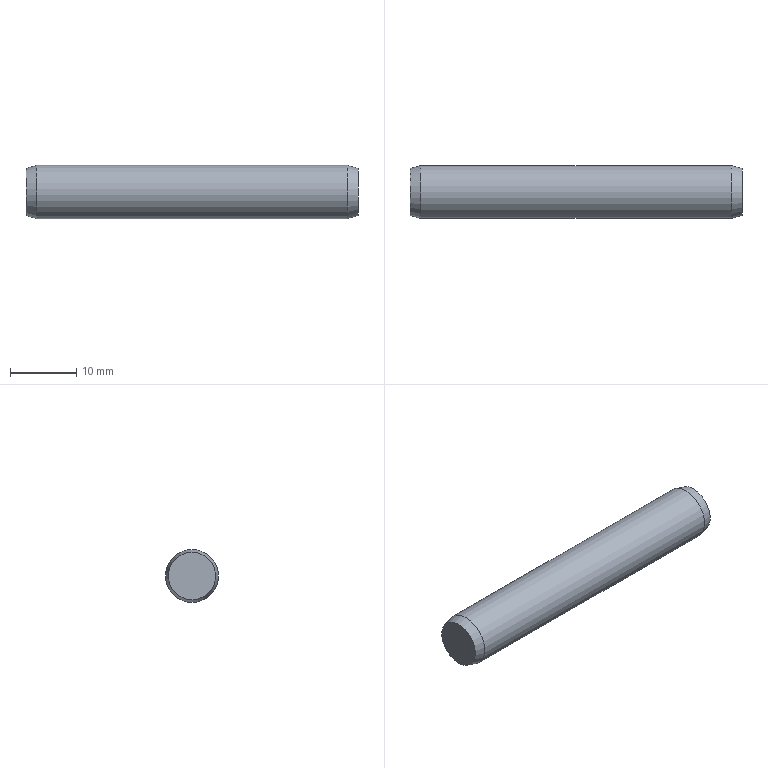Component | NX | GB-T119_1-2000_8X50_2 | 1 solid | 5 faces | box 50 x 8 x 8 mm | volume 2497 mm3 | plane 2 | cone 2 | cylinder 1 | commonest cylinder face diameters 8 x1
STEP:
#1=CARTESIAN_POINT('',(0.,0.,0.));
#2=DIRECTION('',(0.,0.,1.));
#3=DIRECTION('',(1.,0.,0.));
#4=AXIS2_PLACEMENT_3D('',#1,#2,#3);
#5=CARTESIAN_POINT('',(-22.89,40.56,-291.143));
#6=VERTEX_POINT('',#5);
#7=CARTESIAN_POINT('',(-22.89,40.56,-294.714));
#8=DIRECTION('',(-1.,0.,0.));
#9=DIRECTION('',(0.,0.,1.));
#10=AXIS2_PLACEMENT_3D('',#7,#8,#9);
#11=CIRCLE('',#10,3.571);
#12=CARTESIAN_POINT('',(-22.89,40.56,-294.714));
#13=DIRECTION('',(-1.,0.,0.));
#14=DIRECTION('',(0.,0.,1.));
#15=AXIS2_PLACEMENT_3D('',#12,#13,#14);
#16=PLANE('',#15);
#17=CARTESIAN_POINT('',(0.,0.));
#18=DIRECTION('',(1.,0.));
#19=AXIS2_PLACEMENT_2D('',#17,#18);
#20=CIRCLE('',#19,3.571);
#21=(GEOMETRIC_REPRESENTATION_CONTEXT(2)PARAMETRIC_REPRESENTATION_CONTEXT()REPRESENTATION_CONTEXT('',''));
#22=DEFINITIONAL_REPRESENTATION('',(#20),#21);
#23=PCURVE('',#16,#22);
#24=CARTESIAN_POINT('',(-22.89,40.56,-294.714));
#25=DIRECTION('',(1.,0.,0.));
#26=DIRECTION('',(0.,0.,-1.));
#27=AXIS2_PLACEMENT_3D('',#24,#25,#26);
#28=CONICAL_SURFACE('',#27,3.571,0.2618);
#29=CARTESIAN_POINT('',(9.425,-0.));
#30=DIRECTION('',(-1.,0.));
#31=VECTOR('',#30,1.);
#32=LINE('',#29,#31);
#33=(GEOMETRIC_REPRESENTATION_CONTEXT(2)PARAMETRIC_REPRESENTATION_CONTEXT()REPRESENTATION_CONTEXT('',''));
#34=DEFINITIONAL_REPRESENTATION('',(#32),#33);
#35=PCURVE('',#28,#34);
#36=SURFACE_CURVE('',#11,(#23,#35),.PCURVE_S1.);
#37=EDGE_CURVE('',#6,#6,#36,.T.);
#38=ORIENTED_EDGE('',*,*,#37,.T.);
#39=EDGE_LOOP('',(#38));
#40=FACE_BOUND('',#39,.T.);
#41=ADVANCED_FACE('',(#40),#16,.T.);
#42=CARTESIAN_POINT('',(-21.29,40.56,-290.714));
#43=VERTEX_POINT('',#42);
#44=CARTESIAN_POINT('',(-21.29,40.56,-294.714));
#45=DIRECTION('',(-1.,0.,0.));
#46=DIRECTION('',(0.,0.,1.));
#47=AXIS2_PLACEMENT_3D('',#44,#45,#46);
#48=CIRCLE('',#47,4.);
#49=CARTESIAN_POINT('',(9.425,1.6));
#50=DIRECTION('',(-1.,0.));
#51=VECTOR('',#50,1.);
#52=LINE('',#49,#51);
#53=(GEOMETRIC_REPRESENTATION_CONTEXT(2)PARAMETRIC_REPRESENTATION_CONTEXT()REPRESENTATION_CONTEXT('',''));
#54=DEFINITIONAL_REPRESENTATION('',(#52),#53);
#55=PCURVE('',#28,#54);
#56=CARTESIAN_POINT('',(27.11,40.56,-294.714));
#57=DIRECTION('',(-1.,0.,0.));
#58=DIRECTION('',(0.,0.,1.));
#59=AXIS2_PLACEMENT_3D('',#56,#57,#58);
#60=CYLINDRICAL_SURFACE('',#59,4.);
#61=CARTESIAN_POINT('',(0.,48.4));
#62=DIRECTION('',(1.,0.));
#63=VECTOR('',#62,1.);
#64=LINE('',#61,#63);
#65=(GEOMETRIC_REPRESENTATION_CONTEXT(2)PARAMETRIC_REPRESENTATION_CONTEXT()REPRESENTATION_CONTEXT('',''));
#66=DEFINITIONAL_REPRESENTATION('',(#64),#65);
#67=PCURVE('',#60,#66);
#68=SURFACE_CURVE('',#48,(#55,#67),.PCURVE_S1.);
#69=EDGE_CURVE('',#43,#43,#68,.T.);
#70=ORIENTED_EDGE('',*,*,#69,.T.);
#71=CARTESIAN_POINT('',(-22.89,40.56,-291.143));
#72=CARTESIAN_POINT('',(-21.29,40.56,-290.714));
#73=B_SPLINE_CURVE_WITH_KNOTS('',1,(#71,#72),.UNSPECIFIED.,.F.,.F.,(2,2),(-0.,1.656),.PIECEWISE_BEZIER_KNOTS.);
#74=CARTESIAN_POINT('',(3.142,0.));
#75=DIRECTION('',(0.,1.));
#76=VECTOR('',#75,1.);
#77=LINE('',#74,#76);
#78=(GEOMETRIC_REPRESENTATION_CONTEXT(2)PARAMETRIC_REPRESENTATION_CONTEXT()REPRESENTATION_CONTEXT('',''));
#79=DEFINITIONAL_REPRESENTATION('',(#77),#78);
#80=PCURVE('',#28,#79);
#81=CARTESIAN_POINT('',(9.425,0.));
#82=DIRECTION('',(0.,1.));
#83=VECTOR('',#82,1.);
#84=LINE('',#81,#83);
#85=(GEOMETRIC_REPRESENTATION_CONTEXT(2)PARAMETRIC_REPRESENTATION_CONTEXT()REPRESENTATION_CONTEXT('',''));
#86=DEFINITIONAL_REPRESENTATION('',(#84),#85);
#87=PCURVE('',#28,#86);
#88=SEAM_CURVE('',#73,(#80,#87),.PCURVE_S1.);
#89=EDGE_CURVE('',#6,#43,#88,.T.);
#90=ORIENTED_EDGE('',*,*,#89,.F.);
#91=ORIENTED_EDGE('',*,*,#37,.F.);
#92=ORIENTED_EDGE('',*,*,#89,.T.);
#93=EDGE_LOOP('',(#70,#90,#91,#92));
#94=FACE_BOUND('',#93,.T.);
#95=ADVANCED_FACE('',(#94),#28,.T.);
#96=CARTESIAN_POINT('',(25.51,40.56,-290.714));
#97=VERTEX_POINT('',#96);
#98=CARTESIAN_POINT('',(25.51,40.56,-294.714));
#99=DIRECTION('',(-1.,0.,0.));
#100=DIRECTION('',(0.,0.,1.));
#101=AXIS2_PLACEMENT_3D('',#98,#99,#100);
#102=CIRCLE('',#101,4.);
#103=CARTESIAN_POINT('',(0.,1.6));
#104=DIRECTION('',(1.,0.));
#105=VECTOR('',#104,1.);
#106=LINE('',#103,#105);
#107=(GEOMETRIC_REPRESENTATION_CONTEXT(2)PARAMETRIC_REPRESENTATION_CONTEXT()REPRESENTATION_CONTEXT('',''));
#108=DEFINITIONAL_REPRESENTATION('',(#106),#107);
#109=PCURVE('',#60,#108);
#110=CARTESIAN_POINT('',(25.51,40.56,-294.714));
#111=DIRECTION('',(-1.,0.,0.));
#112=DIRECTION('',(0.,0.,1.));
#113=AXIS2_PLACEMENT_3D('',#110,#111,#112);
#114=CONICAL_SURFACE('',#113,4.,0.2618);
#115=CARTESIAN_POINT('',(0.,-0.));
#116=DIRECTION('',(1.,0.));
#117=VECTOR('',#116,1.);
#118=LINE('',#115,#117);
#119=(GEOMETRIC_REPRESENTATION_CONTEXT(2)PARAMETRIC_REPRESENTATION_CONTEXT()REPRESENTATION_CONTEXT('',''));
#120=DEFINITIONAL_REPRESENTATION('',(#118),#119);
#121=PCURVE('',#114,#120);
#122=SURFACE_CURVE('',#102,(#109,#121),.PCURVE_S1.);
#123=EDGE_CURVE('',#97,#97,#122,.T.);
#124=ORIENTED_EDGE('',*,*,#123,.T.);
#125=CARTESIAN_POINT('',(25.51,40.56,-290.714));
#126=CARTESIAN_POINT('',(-21.29,40.56,-290.714));
#127=B_SPLINE_CURVE_WITH_KNOTS('',1,(#125,#126),.UNSPECIFIED.,.F.,.F.,(2,2),(1.6,48.4),.PIECEWISE_BEZIER_KNOTS.);
#128=CARTESIAN_POINT('',(6.283,0.));
#129=DIRECTION('',(0.,1.));
#130=VECTOR('',#129,1.);
#131=LINE('',#128,#130);
#132=(GEOMETRIC_REPRESENTATION_CONTEXT(2)PARAMETRIC_REPRESENTATION_CONTEXT()REPRESENTATION_CONTEXT('',''));
#133=DEFINITIONAL_REPRESENTATION('',(#131),#132);
#134=PCURVE('',#60,#133);
#135=CARTESIAN_POINT('',(0.,0.));
#136=DIRECTION('',(0.,1.));
#137=VECTOR('',#136,1.);
#138=LINE('',#135,#137);
#139=(GEOMETRIC_REPRESENTATION_CONTEXT(2)PARAMETRIC_REPRESENTATION_CONTEXT()REPRESENTATION_CONTEXT('',''));
#140=DEFINITIONAL_REPRESENTATION('',(#138),#139);
#141=PCURVE('',#60,#140);
#142=SEAM_CURVE('',#127,(#134,#141),.PCURVE_S1.);
#143=EDGE_CURVE('',#97,#43,#142,.T.);
#144=ORIENTED_EDGE('',*,*,#143,.T.);
#145=ORIENTED_EDGE('',*,*,#69,.F.);
#146=ORIENTED_EDGE('',*,*,#143,.F.);
#147=EDGE_LOOP('',(#124,#144,#145,#146));
#148=FACE_BOUND('',#147,.T.);
#149=ADVANCED_FACE('',(#148),#60,.T.);
#150=CARTESIAN_POINT('',(27.11,40.56,-291.143));
#151=VERTEX_POINT('',#150);
#152=CARTESIAN_POINT('',(27.11,40.56,-294.714));
#153=DIRECTION('',(-1.,0.,0.));
#154=DIRECTION('',(0.,0.,1.));
#155=AXIS2_PLACEMENT_3D('',#152,#153,#154);
#156=CIRCLE('',#155,3.571);
#157=CARTESIAN_POINT('',(0.,-1.6));
#158=DIRECTION('',(1.,0.));
#159=VECTOR('',#158,1.);
#160=LINE('',#157,#159);
#161=(GEOMETRIC_REPRESENTATION_CONTEXT(2)PARAMETRIC_REPRESENTATION_CONTEXT()REPRESENTATION_CONTEXT('',''));
#162=DEFINITIONAL_REPRESENTATION('',(#160),#161);
#163=PCURVE('',#114,#162);
#164=CARTESIAN_POINT('',(27.11,40.56,-298.285));
#165=DIRECTION('',(1.,0.,0.));
#166=DIRECTION('',(0.,0.,-1.));
#167=AXIS2_PLACEMENT_3D('',#164,#165,#166);
#168=PLANE('',#167);
#169=CARTESIAN_POINT('',(-7.143,0.));
#170=CARTESIAN_POINT('',(-7.143,6.186));
#171=CARTESIAN_POINT('',(-1.786,3.093));
#172=CARTESIAN_POINT('',(3.571,0.));
#173=CARTESIAN_POINT('',(-1.786,-3.093));
#174=CARTESIAN_POINT('',(-7.143,-6.186));
#175=CARTESIAN_POINT('',(-7.143,0.));
#176=(BOUNDED_CURVE()B_SPLINE_CURVE(2,(#169,#170,#171,#172,#173,#174,#175),.UNSPECIFIED.,.T.,.F.)B_SPLINE_CURVE_WITH_KNOTS((1,2,2,2,2,1),(-2.094,0.,2.094,4.189,6.283,8.378),.UNSPECIFIED.)CURVE()GEOMETRIC_REPRESENTATION_ITEM()RATIONAL_B_SPLINE_CURVE((1.,0.5,1.,0.5,1.,0.5,1.))REPRESENTATION_ITEM(''));
#177=(GEOMETRIC_REPRESENTATION_CONTEXT(2)PARAMETRIC_REPRESENTATION_CONTEXT()REPRESENTATION_CONTEXT('',''));
#178=DEFINITIONAL_REPRESENTATION('',(#176),#177);
#179=PCURVE('',#168,#178);
#180=SURFACE_CURVE('',#156,(#163,#179),.PCURVE_S1.);
#181=EDGE_CURVE('',#151,#151,#180,.T.);
#182=ORIENTED_EDGE('',*,*,#181,.T.);
#183=CARTESIAN_POINT('',(27.11,40.56,-291.143));
#184=CARTESIAN_POINT('',(25.51,40.56,-290.714));
#185=B_SPLINE_CURVE_WITH_KNOTS('',1,(#183,#184),.UNSPECIFIED.,.F.,.F.,(2,2),(-1.656,-0.),.PIECEWISE_BEZIER_KNOTS.);
#186=CARTESIAN_POINT('',(6.283,0.));
#187=DIRECTION('',(0.,1.));
#188=VECTOR('',#187,1.);
#189=LINE('',#186,#188);
#190=(GEOMETRIC_REPRESENTATION_CONTEXT(2)PARAMETRIC_REPRESENTATION_CONTEXT()REPRESENTATION_CONTEXT('',''));
#191=DEFINITIONAL_REPRESENTATION('',(#189),#190);
#192=PCURVE('',#114,#191);
#193=CARTESIAN_POINT('',(0.,0.));
#194=DIRECTION('',(0.,1.));
#195=VECTOR('',#194,1.);
#196=LINE('',#193,#195);
#197=(GEOMETRIC_REPRESENTATION_CONTEXT(2)PARAMETRIC_REPRESENTATION_CONTEXT()REPRESENTATION_CONTEXT('',''));
#198=DEFINITIONAL_REPRESENTATION('',(#196),#197);
#199=PCURVE('',#114,#198);
#200=SEAM_CURVE('',#185,(#192,#199),.PCURVE_S1.);
#201=EDGE_CURVE('',#151,#97,#200,.T.);
#202=ORIENTED_EDGE('',*,*,#201,.T.);
#203=ORIENTED_EDGE('',*,*,#123,.F.);
#204=ORIENTED_EDGE('',*,*,#201,.F.);
#205=EDGE_LOOP('',(#182,#202,#203,#204));
#206=FACE_BOUND('',#205,.T.);
#207=ADVANCED_FACE('',(#206),#114,.T.);
#208=ORIENTED_EDGE('',*,*,#181,.F.);
#209=EDGE_LOOP('',(#208));
#210=FACE_BOUND('',#209,.T.);
#211=ADVANCED_FACE('',(#210),#168,.T.);
#212=CLOSED_SHELL('',(#41,#95,#149,#207,#211));
#213=MANIFOLD_SOLID_BREP('',#212);
#214=(LENGTH_UNIT()NAMED_UNIT(*)SI_UNIT(.MILLI.,.METRE.));
#215=UNCERTAINTY_MEASURE_WITH_UNIT(LENGTH_MEASURE(0.00001),#214,'','');
#216=(NAMED_UNIT(*)PLANE_ANGLE_UNIT()SI_UNIT($,.RADIAN.));
#217=(NAMED_UNIT(*)SI_UNIT($,.STERADIAN.)SOLID_ANGLE_UNIT());
#218=(GEOMETRIC_REPRESENTATION_CONTEXT(3)GLOBAL_UNCERTAINTY_ASSIGNED_CONTEXT((#215))GLOBAL_UNIT_ASSIGNED_CONTEXT((#214,#216,#217))REPRESENTATION_CONTEXT('',''));
#219=ADVANCED_BREP_SHAPE_REPRESENTATION('',(#4,#213),#218);